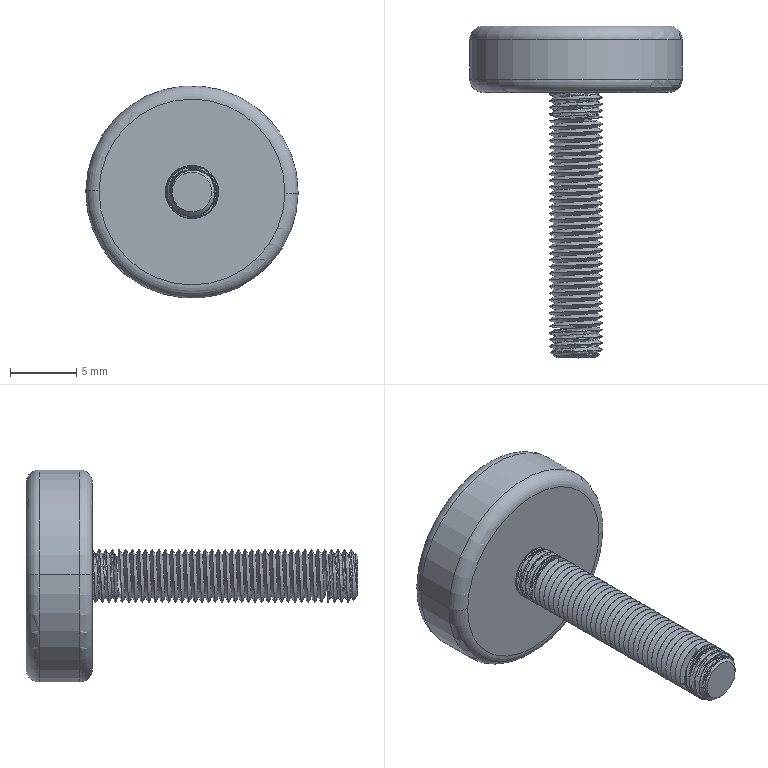Component | SolidWorks | Assembly5.1-1_ShortBoltM4.1-2 | 1 solid | 94 faces | volume 1187 mm3 | cylinder 82 | torus 4 | cone 3 | plane 3 | spline 2 | commonest cylinder face diameters 4 x80 16 x2